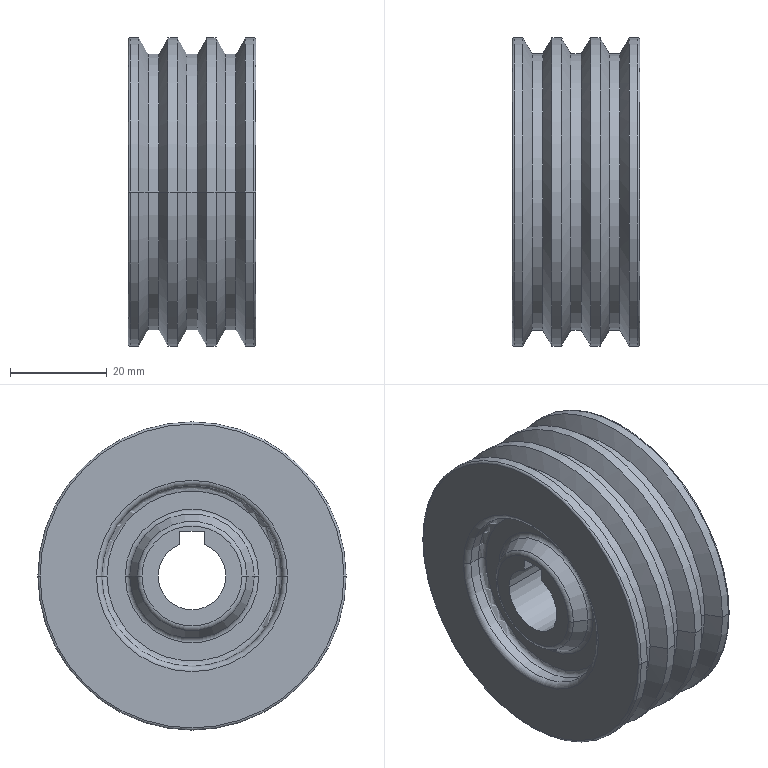Component | SolidWorks | DriveWheel-1 | 1 solid | 66 faces | box 26.4 x 63.8 x 63.8 mm | volume 66255 mm3 | cylinder 21 | torus 20 | cone 16 | plane 9 | commonest cylinder face diameters 63.8 x8 57.2 x6 37.4 x4 14 x3
build123d program:
from build123d import *

# Parameters (mm, degrees)
SCALE1_SCALE       = 0.22
SKETCH2_R          = 7
CUT_EXTRUDE1_DEPTH = 52.975
SKETCH3_W          = 5
SKETCH3_H          = 4.5
CUT_EXTRUDE2_DEPTH = 52.975


with BuildPart() as part:
    # Sketch1 → Revolve Boss (revolve)
    with BuildSketch(Plane(origin=(0, 0, 0), x_dir=(0, 0, -1), z_dir=(1, 0, 0)), mode=Mode.PRIVATE) as revolve_boss_sk:
        with BuildLine():
            Line((-60, 90), (-60, 143))
            ThreePointArc((-60, 143), (-59.414, 144.414), (-58, 145))
            Line((-58, 145), (-50, 145))
            Line((-50, 145), (-41.34, 130))
            Line((-41.34, 130), (-31.34, 130))
            Line((-31.34, 130), (-22.679, 145))
            Line((-22.679, 145), (-13.66, 145))
            Line((-13.66, 145), (-5, 130))
            Line((-5, 130), (5, 130))
            Line((5, 130), (13.66, 145))
            Line((13.66, 145), (22.679, 145))
            Line((22.679, 145), (31.34, 130))
            Line((31.34, 130), (41.34, 130))
            Line((41.34, 130), (50, 145))
            Line((50, 145), (58, 145))
            ThreePointArc((58, 145), (59.414, 144.414), (60, 143))
            Line((60, 143), (60, 90))
            ThreePointArc((60, 90), (58.536, 86.464), (55, 85))
            Line((55, 85), (45, 85))
            ThreePointArc((45, 85), (41.464, 83.536), (40, 80))
            Line((40, 80), (40, 62.887))
            ThreePointArc((40, 62.887), (40.67, 60.387), (42.5, 58.557))
            Line((42.5, 58.557), (54.821, 51.443))
            ThreePointArc((54.821, 51.443), (56.651, 49.613), (57.321, 47.113))
            Line((57.321, 47.113), (57.321, 25))
            Line((57.321, 25), (-57.321, 25))
            Line((-57.321, 25), (-57.321, 47.113))
            ThreePointArc((-57.321, 47.113), (-56.651, 49.613), (-54.821, 51.443))
            Line((-54.821, 51.443), (-42.5, 58.557))
            ThreePointArc((-42.5, 58.557), (-40.67, 60.387), (-40, 62.887))
            Line((-40, 62.887), (-40, 80))
            ThreePointArc((-40, 80), (-41.464, 83.536), (-45, 85))
            Line((-45, 85), (-55, 85))
            ThreePointArc((-55, 85), (-58.536, 86.464), (-60, 90))
        make_face()
    revolve(revolve_boss_sk.sketch.rotate(Axis((0, 0, 0), (0, 0, -1)), 90), axis=Axis((0, 0, 0), (0, 0, -1)))


with BuildPart() as part_1:
    # Scale1: scaled about (0, 0, 0)
    add(part.part.scale(SCALE1_SCALE))

    # Sketch2 → Cut-Extrude1 (cut, through all)
    with BuildSketch(Plane.XY.offset(12.611)):
        Circle(SKETCH2_R)
    extrude(amount=-CUT_EXTRUDE1_DEPTH, mode=Mode.SUBTRACT)

    # Sketch3 → Cut-Extrude2 (cut, through all)
    with BuildSketch(Plane.XY.offset(12.611)):
        with Locations((0, 7)):
            Rectangle(SKETCH3_W, SKETCH3_H)
    extrude(amount=-CUT_EXTRUDE2_DEPTH, mode=Mode.SUBTRACT)


solid = part_1.part

# Placed as in the assembly
solid = solid.moved(Location((28.24, -347.9, 460), (90, -90, 0)))